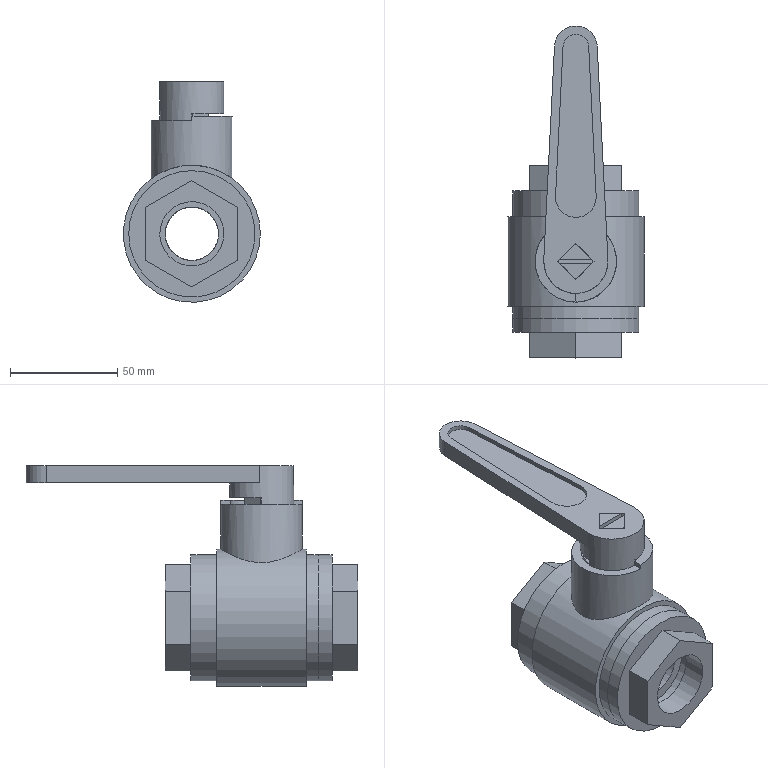Assembly | NX | mm | 9 component files | 9 solids | 143 faces | box 64 x 155 x 103 mm | volume 214814 mm3 | plane 96 | cylinder 42 | sphere 3 | cone 2 | commonest cylinder face diameters 25 x7 35 x4 12 x4 16 x3 59 x3 20 x3 27 x2 34 x2
Bill of materials:
unnamed part 1 | 1 |  | Sphere with a large cylindrical through-bore, two opposite flat faces cut parallel to the bore axis, and an obround (rounded-end) slot cut into the sphere at right angles to the bore.
unnamed part 2 | 1 |  | Stepped, axially symmetric bushing: a hexagonal section, a larger round flange, then a shorter cylindrical spigot with a reduced-diameter groove. A round through-bore runs along the axis.
unnamed part 3 | 1 |  | Tee-shaped body: a horizontal cylindrical main body with a through-bore and slightly raised bands at both ends, a perpendicular cylindrical boss with its own bore, and a smaller polygonal (likely hex) stub at one end.
unnamed part 4 | 1 |  | Plain thick-walled cylindrical ring or sleeve with a concentric through-bore and flat, parallel end faces.
unnamed part 5 | 1 |  | Flat, tapered lever arm with rounded ends. A square through-hole sits in the wider end, set on a cylindrical hub that projects below the arm, and a shallow obround recess or groove runs lengthwise along the top face.
unnamed part 6 | 1 |  | Thick cylindrical ring with a through-bore and two diametrically opposed rectangular slots cut part-way into one end face.
unnamed part 7 | 1 |  | Stepped cylindrical shaft or pin: a larger collar at one end with a chamfer and a flat on its lower portion, a middle round shank, and an end section with two parallel flats and a narrow slot across the end face.
unnamed part 8 | 2 |  | Thin flat ring with a large concentric bore, a fairly narrow radial wall and flat parallel faces.
Mates:
1. fix | ValveBody 1 component
2. concentric | SealRing 2 edge | ValveBody 1 edge
3. concentric | SealRing 1 edge | ValveBonnet 1 edge
4. touch align | ValveCore 1 face | ValveBody 1 face
5. touch align | ValveCore 1 face | ValveBody 1 face
6. concentric | ValveBonnet 1 edge | ValveBody 1 edge
7. touch align | ValveStem 1 face | ValveBody 1
8. concentric | Wrench 1 edge | ValveBody 1 edge
9. touch align | ValveStem 1 face | Wrench 1 face
10. concentric | Gland 1 edge | ValveBody 1
11. concentric | Packing 1 edge | ValveBody 1 edge